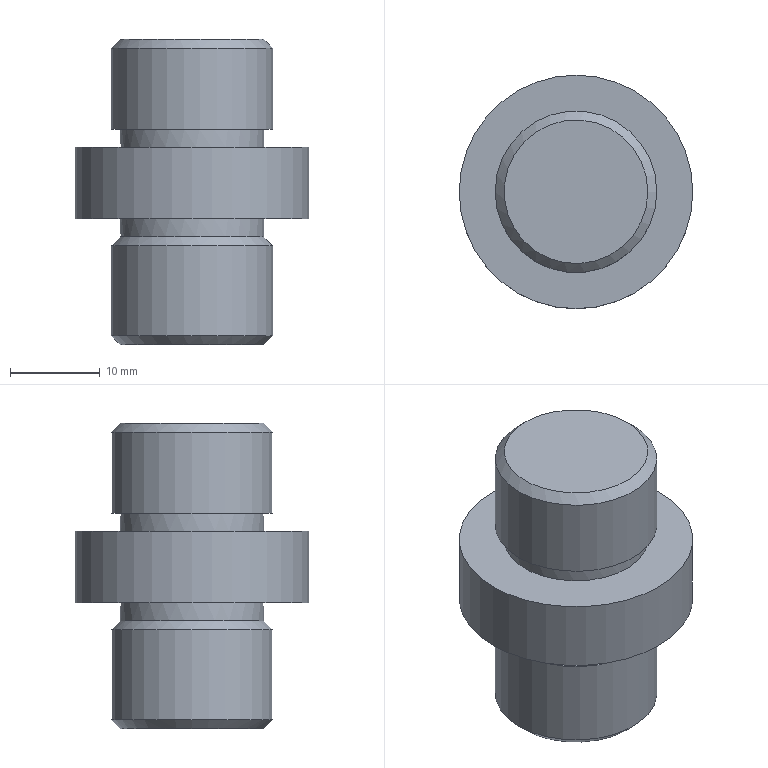Component | NX | DOWEL_PIN | 1 solid | 13 faces | box 26 x 26 x 34 mm | volume 10568 mm3 | plane 5 | cylinder 5 | cone 3 | commonest cylinder face diameters 18 x2 16 x2 26 x1
STEP:
#1=CARTESIAN_POINT('',(0.,0.,0.));
#2=DIRECTION('',(0.,0.,1.));
#3=DIRECTION('',(1.,0.,0.));
#4=AXIS2_PLACEMENT_3D('',#1,#2,#3);
#5=CARTESIAN_POINT('',(-113.,-80.,36.));
#6=VERTEX_POINT('',#5);
#7=CARTESIAN_POINT('',(-105.,-80.,36.));
#8=DIRECTION('',(0.,0.,-1.));
#9=DIRECTION('',(-1.,0.,0.));
#10=AXIS2_PLACEMENT_3D('',#7,#8,#9);
#11=CIRCLE('',#10,8.);
#12=CARTESIAN_POINT('',(-105.,-80.,36.));
#13=DIRECTION('',(0.,0.,-1.));
#14=DIRECTION('',(-1.,0.,0.));
#15=AXIS2_PLACEMENT_3D('',#12,#13,#14);
#16=PLANE('',#15);
#17=CARTESIAN_POINT('',(0.,0.));
#18=DIRECTION('',(1.,0.));
#19=AXIS2_PLACEMENT_2D('',#17,#18);
#20=CIRCLE('',#19,8.);
#21=(GEOMETRIC_REPRESENTATION_CONTEXT(2)PARAMETRIC_REPRESENTATION_CONTEXT()REPRESENTATION_CONTEXT('',''));
#22=DEFINITIONAL_REPRESENTATION('',(#20),#21);
#23=PCURVE('',#16,#22);
#24=CARTESIAN_POINT('',(-105.,-80.,37.));
#25=DIRECTION('',(0.,0.,1.));
#26=DIRECTION('',(1.,0.,0.));
#27=AXIS2_PLACEMENT_3D('',#24,#25,#26);
#28=CONICAL_SURFACE('',#27,9.,0.7854);
#29=CARTESIAN_POINT('',(9.425,-1.));
#30=DIRECTION('',(-1.,0.));
#31=VECTOR('',#30,1.);
#32=LINE('',#29,#31);
#33=(GEOMETRIC_REPRESENTATION_CONTEXT(2)PARAMETRIC_REPRESENTATION_CONTEXT()REPRESENTATION_CONTEXT('',''));
#34=DEFINITIONAL_REPRESENTATION('',(#32),#33);
#35=PCURVE('',#28,#34);
#36=SURFACE_CURVE('',#11,(#23,#35),.PCURVE_S1.);
#37=EDGE_CURVE('',#6,#6,#36,.T.);
#38=ORIENTED_EDGE('',*,*,#37,.T.);
#39=EDGE_LOOP('',(#38));
#40=FACE_BOUND('',#39,.T.);
#41=ADVANCED_FACE('',(#40),#16,.T.);
#42=CARTESIAN_POINT('',(-114.,-80.,37.));
#43=VERTEX_POINT('',#42);
#44=CARTESIAN_POINT('',(-96.,-80.,37.));
#45=VERTEX_POINT('',#44);
#46=CARTESIAN_POINT('',(-105.,-80.,37.));
#47=DIRECTION('',(0.,0.,1.));
#48=DIRECTION('',(-1.,0.,0.));
#49=AXIS2_PLACEMENT_3D('',#46,#47,#48);
#50=CIRCLE('',#49,9.);
#51=CARTESIAN_POINT('',(-105.,-80.,36.));
#52=DIRECTION('',(0.,0.,1.));
#53=DIRECTION('',(1.,0.,0.));
#54=AXIS2_PLACEMENT_3D('',#51,#52,#53);
#55=CYLINDRICAL_SURFACE('',#54,9.);
#56=CARTESIAN_POINT('',(3.142,1.));
#57=DIRECTION('',(1.,0.));
#58=VECTOR('',#57,1.);
#59=LINE('',#56,#58);
#60=(GEOMETRIC_REPRESENTATION_CONTEXT(2)PARAMETRIC_REPRESENTATION_CONTEXT()REPRESENTATION_CONTEXT('',''));
#61=DEFINITIONAL_REPRESENTATION('',(#59),#60);
#62=PCURVE('',#55,#61);
#63=CARTESIAN_POINT('',(3.142,0.));
#64=DIRECTION('',(1.,0.));
#65=VECTOR('',#64,1.);
#66=LINE('',#63,#65);
#67=(GEOMETRIC_REPRESENTATION_CONTEXT(2)PARAMETRIC_REPRESENTATION_CONTEXT()REPRESENTATION_CONTEXT('',''));
#68=DEFINITIONAL_REPRESENTATION('',(#66),#67);
#69=PCURVE('',#28,#68);
#70=SURFACE_CURVE('',#50,(#62,#69),.PCURVE_S1.);
#71=EDGE_CURVE('',#43,#45,#70,.T.);
#72=ORIENTED_EDGE('',*,*,#71,.T.);
#73=CARTESIAN_POINT('',(-96.,-80.,47.));
#74=VERTEX_POINT('',#73);
#75=CARTESIAN_POINT('',(-96.,-80.,37.));
#76=CARTESIAN_POINT('',(-96.,-80.,47.));
#77=B_SPLINE_CURVE_WITH_KNOTS('',1,(#75,#76),.UNSPECIFIED.,.F.,.F.,(2,2),(1.,11.),.PIECEWISE_BEZIER_KNOTS.);
#78=CARTESIAN_POINT('',(6.283,0.));
#79=DIRECTION('',(0.,1.));
#80=VECTOR('',#79,1.);
#81=LINE('',#78,#80);
#82=(GEOMETRIC_REPRESENTATION_CONTEXT(2)PARAMETRIC_REPRESENTATION_CONTEXT()REPRESENTATION_CONTEXT('',''));
#83=DEFINITIONAL_REPRESENTATION('',(#81),#82);
#84=PCURVE('',#55,#83);
#85=CARTESIAN_POINT('',(0.,0.));
#86=DIRECTION('',(0.,1.));
#87=VECTOR('',#86,1.);
#88=LINE('',#85,#87);
#89=(GEOMETRIC_REPRESENTATION_CONTEXT(2)PARAMETRIC_REPRESENTATION_CONTEXT()REPRESENTATION_CONTEXT('',''));
#90=DEFINITIONAL_REPRESENTATION('',(#88),#89);
#91=PCURVE('',#55,#90);
#92=SEAM_CURVE('',#77,(#84,#91),.PCURVE_S1.);
#93=EDGE_CURVE('',#45,#74,#92,.T.);
#94=ORIENTED_EDGE('',*,*,#93,.T.);
#95=CARTESIAN_POINT('',(-105.,-80.,47.));
#96=DIRECTION('',(0.,0.,-1.));
#97=DIRECTION('',(1.,0.,0.));
#98=AXIS2_PLACEMENT_3D('',#95,#96,#97);
#99=CIRCLE('',#98,9.);
#100=CARTESIAN_POINT('',(6.283,11.));
#101=DIRECTION('',(-1.,0.));
#102=VECTOR('',#101,1.);
#103=LINE('',#100,#102);
#104=(GEOMETRIC_REPRESENTATION_CONTEXT(2)PARAMETRIC_REPRESENTATION_CONTEXT()REPRESENTATION_CONTEXT('',''));
#105=DEFINITIONAL_REPRESENTATION('',(#103),#104);
#106=PCURVE('',#55,#105);
#107=CARTESIAN_POINT('',(-105.,-80.,47.));
#108=DIRECTION('',(0.,0.,-1.));
#109=DIRECTION('',(-1.,0.,0.));
#110=AXIS2_PLACEMENT_3D('',#107,#108,#109);
#111=CONICAL_SURFACE('',#110,9.,0.7854);
#112=CARTESIAN_POINT('',(3.142,0.));
#113=DIRECTION('',(1.,0.));
#114=VECTOR('',#113,1.);
#115=LINE('',#112,#114);
#116=(GEOMETRIC_REPRESENTATION_CONTEXT(2)PARAMETRIC_REPRESENTATION_CONTEXT()REPRESENTATION_CONTEXT('',''));
#117=DEFINITIONAL_REPRESENTATION('',(#115),#116);
#118=PCURVE('',#111,#117);
#119=SURFACE_CURVE('',#99,(#106,#118),.PCURVE_S1.);
#120=EDGE_CURVE('',#74,#74,#119,.T.);
#121=ORIENTED_EDGE('',*,*,#120,.T.);
#122=ORIENTED_EDGE('',*,*,#93,.F.);
#123=CARTESIAN_POINT('',(-105.,-80.,37.));
#124=DIRECTION('',(0.,0.,1.));
#125=DIRECTION('',(-1.,0.,0.));
#126=AXIS2_PLACEMENT_3D('',#123,#124,#125);
#127=CIRCLE('',#126,9.);
#128=CARTESIAN_POINT('',(-3.142,1.));
#129=DIRECTION('',(1.,0.));
#130=VECTOR('',#129,1.);
#131=LINE('',#128,#130);
#132=(GEOMETRIC_REPRESENTATION_CONTEXT(2)PARAMETRIC_REPRESENTATION_CONTEXT()REPRESENTATION_CONTEXT('',''));
#133=DEFINITIONAL_REPRESENTATION('',(#131),#132);
#134=PCURVE('',#55,#133);
#135=CARTESIAN_POINT('',(3.142,0.));
#136=DIRECTION('',(1.,0.));
#137=VECTOR('',#136,1.);
#138=LINE('',#135,#137);
#139=(GEOMETRIC_REPRESENTATION_CONTEXT(2)PARAMETRIC_REPRESENTATION_CONTEXT()REPRESENTATION_CONTEXT('',''));
#140=DEFINITIONAL_REPRESENTATION('',(#138),#139);
#141=PCURVE('',#28,#140);
#142=SURFACE_CURVE('',#127,(#134,#141),.PCURVE_S1.);
#143=EDGE_CURVE('',#45,#43,#142,.T.);
#144=ORIENTED_EDGE('',*,*,#143,.T.);
#145=EDGE_LOOP('',(#72,#94,#121,#122,#144));
#146=FACE_BOUND('',#145,.T.);
#147=ADVANCED_FACE('',(#146),#55,.T.);
#148=CARTESIAN_POINT('',(-97.,-80.,50.));
#149=VERTEX_POINT('',#148);
#150=CARTESIAN_POINT('',(-113.,-80.,50.));
#151=VERTEX_POINT('',#150);
#152=CARTESIAN_POINT('',(-105.,-80.,50.));
#153=DIRECTION('',(0.,0.,1.));
#154=DIRECTION('',(-1.,0.,0.));
#155=AXIS2_PLACEMENT_3D('',#152,#153,#154);
#156=CIRCLE('',#155,8.);
#157=CARTESIAN_POINT('',(-105.,-80.,48.));
#158=DIRECTION('',(0.,0.,1.));
#159=DIRECTION('',(1.,0.,0.));
#160=AXIS2_PLACEMENT_3D('',#157,#158,#159);
#161=CYLINDRICAL_SURFACE('',#160,8.);
#162=CARTESIAN_POINT('',(-3.142,2.));
#163=DIRECTION('',(1.,0.));
#164=VECTOR('',#163,1.);
#165=LINE('',#162,#164);
#166=(GEOMETRIC_REPRESENTATION_CONTEXT(2)PARAMETRIC_REPRESENTATION_CONTEXT()REPRESENTATION_CONTEXT('',''));
#167=DEFINITIONAL_REPRESENTATION('',(#165),#166);
#168=PCURVE('',#161,#167);
#169=CARTESIAN_POINT('',(-105.,-80.,50.));
#170=DIRECTION('',(0.,0.,-1.));
#171=DIRECTION('',(-1.,0.,0.));
#172=AXIS2_PLACEMENT_3D('',#169,#170,#171);
#173=PLANE('',#172);
#174=CARTESIAN_POINT('',(8.,0.));
#175=CARTESIAN_POINT('',(8.,-13.856));
#176=CARTESIAN_POINT('',(-4.,-6.928));
#177=CARTESIAN_POINT('',(-16.,-0.));
#178=CARTESIAN_POINT('',(-4.,6.928));
#179=CARTESIAN_POINT('',(8.,13.856));
#180=CARTESIAN_POINT('',(8.,0.));
#181=(BOUNDED_CURVE()B_SPLINE_CURVE(2,(#174,#175,#176,#177,#178,#179,#180),.UNSPECIFIED.,.T.,.F.)B_SPLINE_CURVE_WITH_KNOTS((1,2,2,2,2,1),(-2.094,0.,2.094,4.189,6.283,8.378),.UNSPECIFIED.)CURVE()GEOMETRIC_REPRESENTATION_ITEM()RATIONAL_B_SPLINE_CURVE((1.,0.5,1.,0.5,1.,0.5,1.))REPRESENTATION_ITEM(''));
#182=(GEOMETRIC_REPRESENTATION_CONTEXT(2)PARAMETRIC_REPRESENTATION_CONTEXT()REPRESENTATION_CONTEXT('',''));
#183=DEFINITIONAL_REPRESENTATION('',(#181),#182);
#184=PCURVE('',#173,#183);
#185=SURFACE_CURVE('',#156,(#168,#184),.PCURVE_S1.);
#186=EDGE_CURVE('',#149,#151,#185,.T.);
#187=ORIENTED_EDGE('',*,*,#186,.F.);
#188=CARTESIAN_POINT('',(-97.,-80.,48.));
#189=VERTEX_POINT('',#188);
#190=CARTESIAN_POINT('',(-97.,-80.,48.));
#191=CARTESIAN_POINT('',(-97.,-80.,50.));
#192=B_SPLINE_CURVE_WITH_KNOTS('',1,(#190,#191),.UNSPECIFIED.,.F.,.F.,(2,2),(0.,2.),.PIECEWISE_BEZIER_KNOTS.);
#193=CARTESIAN_POINT('',(0.,0.));
#194=DIRECTION('',(0.,1.));
#195=VECTOR('',#194,1.);
#196=LINE('',#193,#195);
#197=(GEOMETRIC_REPRESENTATION_CONTEXT(2)PARAMETRIC_REPRESENTATION_CONTEXT()REPRESENTATION_CONTEXT('',''));
#198=DEFINITIONAL_REPRESENTATION('',(#196),#197);
#199=PCURVE('',#161,#198);
#200=CARTESIAN_POINT('',(6.283,0.));
#201=DIRECTION('',(0.,1.));
#202=VECTOR('',#201,1.);
#203=LINE('',#200,#202);
#204=(GEOMETRIC_REPRESENTATION_CONTEXT(2)PARAMETRIC_REPRESENTATION_CONTEXT()REPRESENTATION_CONTEXT('',''));
#205=DEFINITIONAL_REPRESENTATION('',(#203),#204);
#206=PCURVE('',#161,#205);
#207=SEAM_CURVE('',#192,(#199,#206),.PCURVE_S1.);
#208=EDGE_CURVE('',#189,#149,#207,.T.);
#209=ORIENTED_EDGE('',*,*,#208,.F.);
#210=CARTESIAN_POINT('',(-105.,-80.,48.));
#211=DIRECTION('',(0.,0.,1.));
#212=DIRECTION('',(1.,0.,0.));
#213=AXIS2_PLACEMENT_3D('',#210,#211,#212);
#214=CIRCLE('',#213,8.);
#215=CARTESIAN_POINT('',(0.,0.));
#216=DIRECTION('',(1.,0.));
#217=VECTOR('',#216,1.);
#218=LINE('',#215,#217);
#219=(GEOMETRIC_REPRESENTATION_CONTEXT(2)PARAMETRIC_REPRESENTATION_CONTEXT()REPRESENTATION_CONTEXT('',''));
#220=DEFINITIONAL_REPRESENTATION('',(#218),#219);
#221=PCURVE('',#161,#220);
#222=CARTESIAN_POINT('',(9.425,-1.));
#223=DIRECTION('',(-1.,0.));
#224=VECTOR('',#223,1.);
#225=LINE('',#222,#224);
#226=(GEOMETRIC_REPRESENTATION_CONTEXT(2)PARAMETRIC_REPRESENTATION_CONTEXT()REPRESENTATION_CONTEXT('',''));
#227=DEFINITIONAL_REPRESENTATION('',(#225),#226);
#228=PCURVE('',#111,#227);
#229=SURFACE_CURVE('',#214,(#221,#228),.PCURVE_S1.);
#230=EDGE_CURVE('',#189,#189,#229,.T.);
#231=ORIENTED_EDGE('',*,*,#230,.T.);
#232=ORIENTED_EDGE('',*,*,#208,.T.);
#233=CARTESIAN_POINT('',(-105.,-80.,50.));
#234=DIRECTION('',(0.,0.,1.));
#235=DIRECTION('',(-1.,0.,0.));
#236=AXIS2_PLACEMENT_3D('',#233,#234,#235);
#237=CIRCLE('',#236,8.);
#238=CARTESIAN_POINT('',(3.142,2.));
#239=DIRECTION('',(1.,0.));
#240=VECTOR('',#239,1.);
#241=LINE('',#238,#240);
#242=(GEOMETRIC_REPRESENTATION_CONTEXT(2)PARAMETRIC_REPRESENTATION_CONTEXT()REPRESENTATION_CONTEXT('',''));
#243=DEFINITIONAL_REPRESENTATION('',(#241),#242);
#244=PCURVE('',#161,#243);
#245=CARTESIAN_POINT('',(8.,0.));
#246=CARTESIAN_POINT('',(8.,-13.856));
#247=CARTESIAN_POINT('',(-4.,-6.928));
#248=CARTESIAN_POINT('',(-16.,-0.));
#249=CARTESIAN_POINT('',(-4.,6.928));
#250=CARTESIAN_POINT('',(8.,13.856));
#251=CARTESIAN_POINT('',(8.,0.));
#252=(BOUNDED_CURVE()B_SPLINE_CURVE(2,(#245,#246,#247,#248,#249,#250,#251),.UNSPECIFIED.,.T.,.F.)B_SPLINE_CURVE_WITH_KNOTS((1,2,2,2,2,1),(-2.094,0.,2.094,4.189,6.283,8.378),.UNSPECIFIED.)CURVE()GEOMETRIC_REPRESENTATION_ITEM()RATIONAL_B_SPLINE_CURVE((1.,0.5,1.,0.5,1.,0.5,1.))REPRESENTATION_ITEM(''));
#253=(GEOMETRIC_REPRESENTATION_CONTEXT(2)PARAMETRIC_REPRESENTATION_CONTEXT()REPRESENTATION_CONTEXT('',''));
#254=DEFINITIONAL_REPRESENTATION('',(#252),#253);
#255=PCURVE('',#173,#254);
#256=SURFACE_CURVE('',#237,(#244,#255),.PCURVE_S1.);
#257=EDGE_CURVE('',#151,#149,#256,.T.);
#258=ORIENTED_EDGE('',*,*,#257,.F.);
#259=EDGE_LOOP('',(#187,#209,#231,#232,#258));
#260=FACE_BOUND('',#259,.T.);
#261=ADVANCED_FACE('',(#260),#161,.T.);
#262=CARTESIAN_POINT('',(-97.,-80.,58.));
#263=VERTEX_POINT('',#262);
#264=CARTESIAN_POINT('',(-105.,-80.,58.));
#265=DIRECTION('',(0.,0.,1.));
#266=DIRECTION('',(1.,0.,0.));
#267=AXIS2_PLACEMENT_3D('',#264,#265,#266);
#268=CIRCLE('',#267,8.);
#269=CARTESIAN_POINT('',(-105.,-80.,58.));
#270=DIRECTION('',(0.,0.,1.));
#271=DIRECTION('',(1.,0.,0.));
#272=AXIS2_PLACEMENT_3D('',#269,#270,#271);
#273=PLANE('',#272);
#274=CARTESIAN_POINT('',(0.,0.));
#275=DIRECTION('',(1.,0.));
#276=AXIS2_PLACEMENT_2D('',#274,#275);
#277=CIRCLE('',#276,8.);
#278=(GEOMETRIC_REPRESENTATION_CONTEXT(2)PARAMETRIC_REPRESENTATION_CONTEXT()REPRESENTATION_CONTEXT('',''));
#279=DEFINITIONAL_REPRESENTATION('',(#277),#278);
#280=PCURVE('',#273,#279);
#281=CARTESIAN_POINT('',(-105.,-80.,58.));
#282=DIRECTION('',(0.,0.,1.));
#283=DIRECTION('',(1.,0.,0.));
#284=AXIS2_PLACEMENT_3D('',#281,#282,#283);
#285=CYLINDRICAL_SURFACE('',#284,8.);
#286=CARTESIAN_POINT('',(0.,0.));
#287=DIRECTION('',(1.,0.));
#288=VECTOR('',#287,1.);
#289=LINE('',#286,#288);
#290=(GEOMETRIC_REPRESENTATION_CONTEXT(2)PARAMETRIC_REPRESENTATION_CONTEXT()REPRESENTATION_CONTEXT('',''));
#291=DEFINITIONAL_REPRESENTATION('',(#289),#290);
#292=PCURVE('',#285,#291);
#293=SURFACE_CURVE('',#268,(#280,#292),.PCURVE_S1.);
#294=EDGE_CURVE('',#263,#263,#293,.T.);
#295=ORIENTED_EDGE('',*,*,#294,.F.);
#296=EDGE_LOOP('',(#295));
#297=FACE_BOUND('',#296,.T.);
#298=CARTESIAN_POINT('',(-92.,-80.,58.));
#299=VERTEX_POINT('',#298);
#300=CARTESIAN_POINT('',(-105.,-80.,58.));
#301=DIRECTION('',(0.,0.,-1.));
#302=DIRECTION('',(1.,0.,0.));
#303=AXIS2_PLACEMENT_3D('',#300,#301,#302);
#304=CIRCLE('',#303,13.);
#305=CARTESIAN_POINT('',(13.,0.));
#306=CARTESIAN_POINT('',(13.,-22.517));
#307=CARTESIAN_POINT('',(-6.5,-11.258));
#308=CARTESIAN_POINT('',(-26.,-0.));
#309=CARTESIAN_POINT('',(-6.5,11.258));
#310=CARTESIAN_POINT('',(13.,22.517));
#311=CARTESIAN_POINT('',(13.,0.));
#312=(BOUNDED_CURVE()B_SPLINE_CURVE(2,(#305,#306,#307,#308,#309,#310,#311),.UNSPECIFIED.,.T.,.F.)B_SPLINE_CURVE_WITH_KNOTS((1,2,2,2,2,1),(-2.094,0.,2.094,4.189,6.283,8.378),.UNSPECIFIED.)CURVE()GEOMETRIC_REPRESENTATION_ITEM()RATIONAL_B_SPLINE_CURVE((1.,0.5,1.,0.5,1.,0.5,1.))REPRESENTATION_ITEM(''));
#313=(GEOMETRIC_REPRESENTATION_CONTEXT(2)PARAMETRIC_REPRESENTATION_CONTEXT()REPRESENTATION_CONTEXT('',''));
#314=DEFINITIONAL_REPRESENTATION('',(#312),#313);
#315=PCURVE('',#273,#314);
#316=CARTESIAN_POINT('',(-105.,-80.,50.));
#317=DIRECTION('',(0.,0.,1.));
#318=DIRECTION('',(1.,0.,0.));
#319=AXIS2_PLACEMENT_3D('',#316,#317,#318);
#320=CYLINDRICAL_SURFACE('',#319,13.);
#321=CARTESIAN_POINT('',(6.283,8.));
#322=DIRECTION('',(-1.,0.));
#323=VECTOR('',#322,1.);
#324=LINE('',#321,#323);
#325=(GEOMETRIC_REPRESENTATION_CONTEXT(2)PARAMETRIC_REPRESENTATION_CONTEXT()REPRESENTATION_CONTEXT('',''));
#326=DEFINITIONAL_REPRESENTATION('',(#324),#325);
#327=PCURVE('',#320,#326);
#328=SURFACE_CURVE('',#304,(#315,#327),.PCURVE_S1.);
#329=EDGE_CURVE('',#299,#299,#328,.T.);
#330=ORIENTED_EDGE('',*,*,#329,.F.);
#331=EDGE_LOOP('',(#330));
#332=FACE_BOUND('',#331,.T.);
#333=ADVANCED_FACE('',(#297,#332),#273,.T.);
#334=ORIENTED_EDGE('',*,*,#257,.T.);
#335=ORIENTED_EDGE('',*,*,#186,.T.);
#336=EDGE_LOOP('',(#334,#335));
#337=FACE_BOUND('',#336,.T.);
#338=CARTESIAN_POINT('',(-92.,-80.,50.));
#339=VERTEX_POINT('',#338);
#340=CARTESIAN_POINT('',(-105.,-80.,50.));
#341=DIRECTION('',(0.,0.,1.));
#342=DIRECTION('',(1.,0.,0.));
#343=AXIS2_PLACEMENT_3D('',#340,#341,#342);
#344=CIRCLE('',#343,13.);
#345=CARTESIAN_POINT('',(-13.,0.));
#346=CARTESIAN_POINT('',(-13.,22.517));
#347=CARTESIAN_POINT('',(6.5,11.258));
#348=CARTESIAN_POINT('',(26.,0.));
#349=CARTESIAN_POINT('',(6.5,-11.258));
#350=CARTESIAN_POINT('',(-13.,-22.517));
#351=CARTESIAN_POINT('',(-13.,0.));
#352=(BOUNDED_CURVE()B_SPLINE_CURVE(2,(#345,#346,#347,#348,#349,#350,#351),.UNSPECIFIED.,.T.,.F.)B_SPLINE_CURVE_WITH_KNOTS((1,2,2,2,2,1),(-2.094,0.,2.094,4.189,6.283,8.378),.UNSPECIFIED.)CURVE()GEOMETRIC_REPRESENTATION_ITEM()RATIONAL_B_SPLINE_CURVE((1.,0.5,1.,0.5,1.,0.5,1.))REPRESENTATION_ITEM(''));
#353=(GEOMETRIC_REPRESENTATION_CONTEXT(2)PARAMETRIC_REPRESENTATION_CONTEXT()REPRESENTATION_CONTEXT('',''));
#354=DEFINITIONAL_REPRESENTATION('',(#352),#353);
#355=PCURVE('',#173,#354);
#356=CARTESIAN_POINT('',(0.,0.));
#357=DIRECTION('',(1.,0.));
#358=VECTOR('',#357,1.);
#359=LINE('',#356,#358);
#360=(GEOMETRIC_REPRESENTATION_CONTEXT(2)PARAMETRIC_REPRESENTATION_CONTEXT()REPRESENTATION_CONTEXT('',''));
#361=DEFINITIONAL_REPRESENTATION('',(#359),#360);
#362=PCURVE('',#320,#361);
#363=SURFACE_CURVE('',#344,(#355,#362),.PCURVE_S1.);
#364=EDGE_CURVE('',#339,#339,#363,.T.);
#365=ORIENTED_EDGE('',*,*,#364,.F.);
#366=EDGE_LOOP('',(#365));
#367=FACE_BOUND('',#366,.T.);
#368=ADVANCED_FACE('',(#337,#367),#173,.T.);
#369=ORIENTED_EDGE('',*,*,#329,.T.);
#370=CARTESIAN_POINT('',(-92.,-80.,50.));
#371=CARTESIAN_POINT('',(-92.,-80.,58.));
#372=B_SPLINE_CURVE_WITH_KNOTS('',1,(#370,#371),.UNSPECIFIED.,.F.,.F.,(2,2),(0.,8.),.PIECEWISE_BEZIER_KNOTS.);
#373=CARTESIAN_POINT('',(0.,0.));
#374=DIRECTION('',(0.,1.));
#375=VECTOR('',#374,1.);
#376=LINE('',#373,#375);
#377=(GEOMETRIC_REPRESENTATION_CONTEXT(2)PARAMETRIC_REPRESENTATION_CONTEXT()REPRESENTATION_CONTEXT('',''));
#378=DEFINITIONAL_REPRESENTATION('',(#376),#377);
#379=PCURVE('',#320,#378);
#380=CARTESIAN_POINT('',(6.283,0.));
#381=DIRECTION('',(0.,1.));
#382=VECTOR('',#381,1.);
#383=LINE('',#380,#382);
#384=(GEOMETRIC_REPRESENTATION_CONTEXT(2)PARAMETRIC_REPRESENTATION_CONTEXT()REPRESENTATION_CONTEXT('',''));
#385=DEFINITIONAL_REPRESENTATION('',(#383),#384);
#386=PCURVE('',#320,#385);
#387=SEAM_CURVE('',#372,(#379,#386),.PCURVE_S1.);
#388=EDGE_CURVE('',#339,#299,#387,.T.);
#389=ORIENTED_EDGE('',*,*,#388,.F.);
#390=ORIENTED_EDGE('',*,*,#364,.T.);
#391=ORIENTED_EDGE('',*,*,#388,.T.);
#392=EDGE_LOOP('',(#369,#389,#390,#391));
#393=FACE_BOUND('',#392,.T.);
#394=ADVANCED_FACE('',(#393),#320,.T.);
#395=CARTESIAN_POINT('',(-97.,-80.,60.));
#396=VERTEX_POINT('',#395);
#397=CARTESIAN_POINT('',(-113.,-80.,60.));
#398=VERTEX_POINT('',#397);
#399=CARTESIAN_POINT('',(-105.,-80.,60.));
#400=DIRECTION('',(0.,0.,1.));
#401=DIRECTION('',(-1.,0.,0.));
#402=AXIS2_PLACEMENT_3D('',#399,#400,#401);
#403=CIRCLE('',#402,8.);
#404=CARTESIAN_POINT('',(-3.142,2.));
#405=DIRECTION('',(1.,0.));
#406=VECTOR('',#405,1.);
#407=LINE('',#404,#406);
#408=(GEOMETRIC_REPRESENTATION_CONTEXT(2)PARAMETRIC_REPRESENTATION_CONTEXT()REPRESENTATION_CONTEXT('',''));
#409=DEFINITIONAL_REPRESENTATION('',(#407),#408);
#410=PCURVE('',#285,#409);
#411=CARTESIAN_POINT('',(-105.,-80.,60.));
#412=DIRECTION('',(0.,0.,-1.));
#413=DIRECTION('',(-1.,0.,0.));
#414=AXIS2_PLACEMENT_3D('',#411,#412,#413);
#415=PLANE('',#414);
#416=CARTESIAN_POINT('',(8.,0.));
#417=CARTESIAN_POINT('',(8.,-13.856));
#418=CARTESIAN_POINT('',(-4.,-6.928));
#419=CARTESIAN_POINT('',(-16.,-0.));
#420=CARTESIAN_POINT('',(-4.,6.928));
#421=CARTESIAN_POINT('',(8.,13.856));
#422=CARTESIAN_POINT('',(8.,0.));
#423=(BOUNDED_CURVE()B_SPLINE_CURVE(2,(#416,#417,#418,#419,#420,#421,#422),.UNSPECIFIED.,.T.,.F.)B_SPLINE_CURVE_WITH_KNOTS((1,2,2,2,2,1),(-2.094,0.,2.094,4.189,6.283,8.378),.UNSPECIFIED.)CURVE()GEOMETRIC_REPRESENTATION_ITEM()RATIONAL_B_SPLINE_CURVE((1.,0.5,1.,0.5,1.,0.5,1.))REPRESENTATION_ITEM(''));
#424=(GEOMETRIC_REPRESENTATION_CONTEXT(2)PARAMETRIC_REPRESENTATION_CONTEXT()REPRESENTATION_CONTEXT('',''));
#425=DEFINITIONAL_REPRESENTATION('',(#423),#424);
#426=PCURVE('',#415,#425);
#427=SURFACE_CURVE('',#403,(#410,#426),.PCURVE_S1.);
#428=EDGE_CURVE('',#396,#398,#427,.T.);
#429=ORIENTED_EDGE('',*,*,#428,.F.);
#430=CARTESIAN_POINT('',(-97.,-80.,58.));
#431=CARTESIAN_POINT('',(-97.,-80.,60.));
#432=B_SPLINE_CURVE_WITH_KNOTS('',1,(#430,#431),.UNSPECIFIED.,.F.,.F.,(2,2),(0.,2.),.PIECEWISE_BEZIER_KNOTS.);
#433=CARTESIAN_POINT('',(0.,0.));
#434=DIRECTION('',(0.,1.));
#435=VECTOR('',#434,1.);
#436=LINE('',#433,#435);
#437=(GEOMETRIC_REPRESENTATION_CONTEXT(2)PARAMETRIC_REPRESENTATION_CONTEXT()REPRESENTATION_CONTEXT('',''));
#438=DEFINITIONAL_REPRESENTATION('',(#436),#437);
#439=PCURVE('',#285,#438);
#440=CARTESIAN_POINT('',(6.283,0.));
#441=DIRECTION('',(0.,1.));
#442=VECTOR('',#441,1.);
#443=LINE('',#440,#442);
#444=(GEOMETRIC_REPRESENTATION_CONTEXT(2)PARAMETRIC_REPRESENTATION_CONTEXT()REPRESENTATION_CONTEXT('',''));
#445=DEFINITIONAL_REPRESENTATION('',(#443),#444);
#446=PCURVE('',#285,#445);
#447=SEAM_CURVE('',#432,(#439,#446),.PCURVE_S1.);
#448=EDGE_CURVE('',#263,#396,#447,.T.);
#449=ORIENTED_EDGE('',*,*,#448,.F.);
#450=ORIENTED_EDGE('',*,*,#294,.T.);
#451=ORIENTED_EDGE('',*,*,#448,.T.);
#452=CARTESIAN_POINT('',(-105.,-80.,60.));
#453=DIRECTION('',(0.,0.,1.));
#454=DIRECTION('',(-1.,0.,0.));
#455=AXIS2_PLACEMENT_3D('',#452,#453,#454);
#456=CIRCLE('',#455,8.);
#457=CARTESIAN_POINT('',(3.142,2.));
#458=DIRECTION('',(1.,0.));
#459=VECTOR('',#458,1.);
#460=LINE('',#457,#459);
#461=(GEOMETRIC_REPRESENTATION_CONTEXT(2)PARAMETRIC_REPRESENTATION_CONTEXT()REPRESENTATION_CONTEXT('',''));
#462=DEFINITIONAL_REPRESENTATION('',(#460),#461);
#463=PCURVE('',#285,#462);
#464=CARTESIAN_POINT('',(8.,0.));
#465=CARTESIAN_POINT('',(8.,-13.856));
#466=CARTESIAN_POINT('',(-4.,-6.928));
#467=CARTESIAN_POINT('',(-16.,-0.));
#468=CARTESIAN_POINT('',(-4.,6.928));
#469=CARTESIAN_POINT('',(8.,13.856));
#470=CARTESIAN_POINT('',(8.,0.));
#471=(BOUNDED_CURVE()B_SPLINE_CURVE(2,(#464,#465,#466,#467,#468,#469,#470),.UNSPECIFIED.,.T.,.F.)B_SPLINE_CURVE_WITH_KNOTS((1,2,2,2,2,1),(-2.094,0.,2.094,4.189,6.283,8.378),.UNSPECIFIED.)CURVE()GEOMETRIC_REPRESENTATION_ITEM()RATIONAL_B_SPLINE_CURVE((1.,0.5,1.,0.5,1.,0.5,1.))REPRESENTATION_ITEM(''));
#472=(GEOMETRIC_REPRESENTATION_CONTEXT(2)PARAMETRIC_REPRESENTATION_CONTEXT()REPRESENTATION_CONTEXT('',''));
#473=DEFINITIONAL_REPRESENTATION('',(#471),#472);
#474=PCURVE('',#415,#473);
#475=SURFACE_CURVE('',#456,(#463,#474),.PCURVE_S1.);
#476=EDGE_CURVE('',#398,#396,#475,.T.);
#477=ORIENTED_EDGE('',*,*,#476,.F.);
#478=EDGE_LOOP('',(#429,#449,#450,#451,#477));
#479=FACE_BOUND('',#478,.T.);
#480=ADVANCED_FACE('',(#479),#285,.T.);
#481=CARTESIAN_POINT('',(-97.,-80.,70.));
#482=VERTEX_POINT('',#481);
#483=CARTESIAN_POINT('',(-105.,-80.,70.));
#484=DIRECTION('',(0.,0.,1.));
#485=DIRECTION('',(1.,0.,0.));
#486=AXIS2_PLACEMENT_3D('',#483,#484,#485);
#487=CIRCLE('',#486,8.);
#488=CARTESIAN_POINT('',(-105.,-80.,70.));
#489=DIRECTION('',(0.,0.,1.));
#490=DIRECTION('',(1.,0.,0.));
#491=AXIS2_PLACEMENT_3D('',#488,#489,#490);
#492=PLANE('',#491);
#493=CARTESIAN_POINT('',(0.,0.));
#494=DIRECTION('',(1.,0.));
#495=AXIS2_PLACEMENT_2D('',#493,#494);
#496=CIRCLE('',#495,8.);
#497=(GEOMETRIC_REPRESENTATION_CONTEXT(2)PARAMETRIC_REPRESENTATION_CONTEXT()REPRESENTATION_CONTEXT('',''));
#498=DEFINITIONAL_REPRESENTATION('',(#496),#497);
#499=PCURVE('',#492,#498);
#500=CARTESIAN_POINT('',(-105.,-80.,69.));
#501=DIRECTION('',(0.,0.,-1.));
#502=DIRECTION('',(-1.,0.,0.));
#503=AXIS2_PLACEMENT_3D('',#500,#501,#502);
#504=CONICAL_SURFACE('',#503,9.,0.7854);
#505=CARTESIAN_POINT('',(9.425,-1.));
#506=DIRECTION('',(-1.,0.));
#507=VECTOR('',#506,1.);
#508=LINE('',#505,#507);
#509=(GEOMETRIC_REPRESENTATION_CONTEXT(2)PARAMETRIC_REPRESENTATION_CONTEXT()REPRESENTATION_CONTEXT('',''));
#510=DEFINITIONAL_REPRESENTATION('',(#508),#509);
#511=PCURVE('',#504,#510);
#512=SURFACE_CURVE('',#487,(#499,#511),.PCURVE_S1.);
#513=EDGE_CURVE('',#482,#482,#512,.T.);
#514=ORIENTED_EDGE('',*,*,#513,.T.);
#515=EDGE_LOOP('',(#514));
#516=FACE_BOUND('',#515,.T.);
#517=ADVANCED_FACE('',(#516),#492,.T.);
#518=ORIENTED_EDGE('',*,*,#476,.T.);
#519=ORIENTED_EDGE('',*,*,#428,.T.);
#520=EDGE_LOOP('',(#518,#519));
#521=FACE_BOUND('',#520,.T.);
#522=CARTESIAN_POINT('',(-96.,-80.,60.));
#523=VERTEX_POINT('',#522);
#524=CARTESIAN_POINT('',(-105.,-80.,60.));
#525=DIRECTION('',(0.,0.,1.));
#526=DIRECTION('',(1.,0.,0.));
#527=AXIS2_PLACEMENT_3D('',#524,#525,#526);
#528=CIRCLE('',#527,9.);
#529=CARTESIAN_POINT('',(-9.,0.));
#530=CARTESIAN_POINT('',(-9.,15.588));
#531=CARTESIAN_POINT('',(4.5,7.794));
#532=CARTESIAN_POINT('',(18.,0.));
#533=CARTESIAN_POINT('',(4.5,-7.794));
#534=CARTESIAN_POINT('',(-9.,-15.588));
#535=CARTESIAN_POINT('',(-9.,0.));
#536=(BOUNDED_CURVE()B_SPLINE_CURVE(2,(#529,#530,#531,#532,#533,#534,#535),.UNSPECIFIED.,.T.,.F.)B_SPLINE_CURVE_WITH_KNOTS((1,2,2,2,2,1),(-2.094,0.,2.094,4.189,6.283,8.378),.UNSPECIFIED.)CURVE()GEOMETRIC_REPRESENTATION_ITEM()RATIONAL_B_SPLINE_CURVE((1.,0.5,1.,0.5,1.,0.5,1.))REPRESENTATION_ITEM(''));
#537=(GEOMETRIC_REPRESENTATION_CONTEXT(2)PARAMETRIC_REPRESENTATION_CONTEXT()REPRESENTATION_CONTEXT('',''));
#538=DEFINITIONAL_REPRESENTATION('',(#536),#537);
#539=PCURVE('',#415,#538);
#540=CARTESIAN_POINT('',(-105.,-80.,60.));
#541=DIRECTION('',(0.,0.,1.));
#542=DIRECTION('',(1.,0.,0.));
#543=AXIS2_PLACEMENT_3D('',#540,#541,#542);
#544=CYLINDRICAL_SURFACE('',#543,9.);
#545=CARTESIAN_POINT('',(0.,0.));
#546=DIRECTION('',(1.,0.));
#547=VECTOR('',#546,1.);
#548=LINE('',#545,#547);
#549=(GEOMETRIC_REPRESENTATION_CONTEXT(2)PARAMETRIC_REPRESENTATION_CONTEXT()REPRESENTATION_CONTEXT('',''));
#550=DEFINITIONAL_REPRESENTATION('',(#548),#549);
#551=PCURVE('',#544,#550);
#552=SURFACE_CURVE('',#528,(#539,#551),.PCURVE_S1.);
#553=EDGE_CURVE('',#523,#523,#552,.T.);
#554=ORIENTED_EDGE('',*,*,#553,.F.);
#555=EDGE_LOOP('',(#554));
#556=FACE_BOUND('',#555,.T.);
#557=ADVANCED_FACE('',(#521,#556),#415,.T.);
#558=CARTESIAN_POINT('',(-96.,-80.,69.));
#559=VERTEX_POINT('',#558);
#560=CARTESIAN_POINT('',(-105.,-80.,69.));
#561=DIRECTION('',(0.,0.,-1.));
#562=DIRECTION('',(1.,0.,0.));
#563=AXIS2_PLACEMENT_3D('',#560,#561,#562);
#564=CIRCLE('',#563,9.);
#565=CARTESIAN_POINT('',(6.283,9.));
#566=DIRECTION('',(-1.,0.));
#567=VECTOR('',#566,1.);
#568=LINE('',#565,#567);
#569=(GEOMETRIC_REPRESENTATION_CONTEXT(2)PARAMETRIC_REPRESENTATION_CONTEXT()REPRESENTATION_CONTEXT('',''));
#570=DEFINITIONAL_REPRESENTATION('',(#568),#569);
#571=PCURVE('',#544,#570);
#572=CARTESIAN_POINT('',(3.142,0.));
#573=DIRECTION('',(1.,0.));
#574=VECTOR('',#573,1.);
#575=LINE('',#572,#574);
#576=(GEOMETRIC_REPRESENTATION_CONTEXT(2)PARAMETRIC_REPRESENTATION_CONTEXT()REPRESENTATION_CONTEXT('',''));
#577=DEFINITIONAL_REPRESENTATION('',(#575),#576);
#578=PCURVE('',#504,#577);
#579=SURFACE_CURVE('',#564,(#571,#578),.PCURVE_S1.);
#580=EDGE_CURVE('',#559,#559,#579,.T.);
#581=ORIENTED_EDGE('',*,*,#580,.T.);
#582=CARTESIAN_POINT('',(-96.,-80.,60.));
#583=CARTESIAN_POINT('',(-96.,-80.,69.));
#584=B_SPLINE_CURVE_WITH_KNOTS('',1,(#582,#583),.UNSPECIFIED.,.F.,.F.,(2,2),(0.,9.),.PIECEWISE_BEZIER_KNOTS.);
#585=CARTESIAN_POINT('',(0.,0.));
#586=DIRECTION('',(0.,1.));
#587=VECTOR('',#586,1.);
#588=LINE('',#585,#587);
#589=(GEOMETRIC_REPRESENTATION_CONTEXT(2)PARAMETRIC_REPRESENTATION_CONTEXT()REPRESENTATION_CONTEXT('',''));
#590=DEFINITIONAL_REPRESENTATION('',(#588),#589);
#591=PCURVE('',#544,#590);
#592=CARTESIAN_POINT('',(6.283,0.));
#593=DIRECTION('',(0.,1.));
#594=VECTOR('',#593,1.);
#595=LINE('',#592,#594);
#596=(GEOMETRIC_REPRESENTATION_CONTEXT(2)PARAMETRIC_REPRESENTATION_CONTEXT()REPRESENTATION_CONTEXT('',''));
#597=DEFINITIONAL_REPRESENTATION('',(#595),#596);
#598=PCURVE('',#544,#597);
#599=SEAM_CURVE('',#584,(#591,#598),.PCURVE_S1.);
#600=EDGE_CURVE('',#523,#559,#599,.T.);
#601=ORIENTED_EDGE('',*,*,#600,.F.);
#602=ORIENTED_EDGE('',*,*,#553,.T.);
#603=ORIENTED_EDGE('',*,*,#600,.T.);
#604=EDGE_LOOP('',(#581,#601,#602,#603));
#605=FACE_BOUND('',#604,.T.);
#606=ADVANCED_FACE('',(#605),#544,.T.);
#607=ORIENTED_EDGE('',*,*,#37,.F.);
#608=CARTESIAN_POINT('',(-113.,-80.,36.));
#609=CARTESIAN_POINT('',(-114.,-80.,37.));
#610=B_SPLINE_CURVE_WITH_KNOTS('',1,(#608,#609),.UNSPECIFIED.,.F.,.F.,(2,2),(-1.414,0.),.PIECEWISE_BEZIER_KNOTS.);
#611=CARTESIAN_POINT('',(9.425,0.));
#612=DIRECTION('',(0.,1.));
#613=VECTOR('',#612,1.);
#614=LINE('',#611,#613);
#615=(GEOMETRIC_REPRESENTATION_CONTEXT(2)PARAMETRIC_REPRESENTATION_CONTEXT()REPRESENTATION_CONTEXT('',''));
#616=DEFINITIONAL_REPRESENTATION('',(#614),#615);
#617=PCURVE('',#28,#616);
#618=CARTESIAN_POINT('',(3.142,0.));
#619=DIRECTION('',(0.,1.));
#620=VECTOR('',#619,1.);
#621=LINE('',#618,#620);
#622=(GEOMETRIC_REPRESENTATION_CONTEXT(2)PARAMETRIC_REPRESENTATION_CONTEXT()REPRESENTATION_CONTEXT('',''));
#623=DEFINITIONAL_REPRESENTATION('',(#621),#622);
#624=PCURVE('',#28,#623);
#625=SEAM_CURVE('',#610,(#617,#624),.PCURVE_S1.);
#626=EDGE_CURVE('',#6,#43,#625,.T.);
#627=ORIENTED_EDGE('',*,*,#626,.T.);
#628=ORIENTED_EDGE('',*,*,#143,.F.);
#629=ORIENTED_EDGE('',*,*,#71,.F.);
#630=ORIENTED_EDGE('',*,*,#626,.F.);
#631=EDGE_LOOP('',(#607,#627,#628,#629,#630));
#632=FACE_BOUND('',#631,.T.);
#633=ADVANCED_FACE('',(#632),#28,.T.);
#634=ORIENTED_EDGE('',*,*,#230,.F.);
#635=CARTESIAN_POINT('',(-97.,-80.,48.));
#636=CARTESIAN_POINT('',(-96.,-80.,47.));
#637=B_SPLINE_CURVE_WITH_KNOTS('',1,(#635,#636),.UNSPECIFIED.,.F.,.F.,(2,2),(-1.414,0.),.PIECEWISE_BEZIER_KNOTS.);
#638=CARTESIAN_POINT('',(9.425,0.));
#639=DIRECTION('',(0.,1.));
#640=VECTOR('',#639,1.);
#641=LINE('',#638,#640);
#642=(GEOMETRIC_REPRESENTATION_CONTEXT(2)PARAMETRIC_REPRESENTATION_CONTEXT()REPRESENTATION_CONTEXT('',''));
#643=DEFINITIONAL_REPRESENTATION('',(#641),#642);
#644=PCURVE('',#111,#643);
#645=CARTESIAN_POINT('',(3.142,0.));
#646=DIRECTION('',(0.,1.));
#647=VECTOR('',#646,1.);
#648=LINE('',#645,#647);
#649=(GEOMETRIC_REPRESENTATION_CONTEXT(2)PARAMETRIC_REPRESENTATION_CONTEXT()REPRESENTATION_CONTEXT('',''));
#650=DEFINITIONAL_REPRESENTATION('',(#648),#649);
#651=PCURVE('',#111,#650);
#652=SEAM_CURVE('',#637,(#644,#651),.PCURVE_S1.);
#653=EDGE_CURVE('',#189,#74,#652,.T.);
#654=ORIENTED_EDGE('',*,*,#653,.T.);
#655=ORIENTED_EDGE('',*,*,#120,.F.);
#656=ORIENTED_EDGE('',*,*,#653,.F.);
#657=EDGE_LOOP('',(#634,#654,#655,#656));
#658=FACE_BOUND('',#657,.T.);
#659=ADVANCED_FACE('',(#658),#111,.T.);
#660=ORIENTED_EDGE('',*,*,#513,.F.);
#661=CARTESIAN_POINT('',(-97.,-80.,70.));
#662=CARTESIAN_POINT('',(-96.,-80.,69.));
#663=B_SPLINE_CURVE_WITH_KNOTS('',1,(#661,#662),.UNSPECIFIED.,.F.,.F.,(2,2),(-1.414,0.),.PIECEWISE_BEZIER_KNOTS.);
#664=CARTESIAN_POINT('',(9.425,0.));
#665=DIRECTION('',(0.,1.));
#666=VECTOR('',#665,1.);
#667=LINE('',#664,#666);
#668=(GEOMETRIC_REPRESENTATION_CONTEXT(2)PARAMETRIC_REPRESENTATION_CONTEXT()REPRESENTATION_CONTEXT('',''));
#669=DEFINITIONAL_REPRESENTATION('',(#667),#668);
#670=PCURVE('',#504,#669);
#671=CARTESIAN_POINT('',(3.142,0.));
#672=DIRECTION('',(0.,1.));
#673=VECTOR('',#672,1.);
#674=LINE('',#671,#673);
#675=(GEOMETRIC_REPRESENTATION_CONTEXT(2)PARAMETRIC_REPRESENTATION_CONTEXT()REPRESENTATION_CONTEXT('',''));
#676=DEFINITIONAL_REPRESENTATION('',(#674),#675);
#677=PCURVE('',#504,#676);
#678=SEAM_CURVE('',#663,(#670,#677),.PCURVE_S1.);
#679=EDGE_CURVE('',#482,#559,#678,.T.);
#680=ORIENTED_EDGE('',*,*,#679,.T.);
#681=ORIENTED_EDGE('',*,*,#580,.F.);
#682=ORIENTED_EDGE('',*,*,#679,.F.);
#683=EDGE_LOOP('',(#660,#680,#681,#682));
#684=FACE_BOUND('',#683,.T.);
#685=ADVANCED_FACE('',(#684),#504,.T.);
#686=CLOSED_SHELL('',(#41,#147,#261,#333,#368,#394,#480,#517,#557,#606,#633,#659,#685));
#687=MANIFOLD_SOLID_BREP('',#686);
#688=(LENGTH_UNIT()NAMED_UNIT(*)SI_UNIT(.MILLI.,.METRE.));
#689=UNCERTAINTY_MEASURE_WITH_UNIT(LENGTH_MEASURE(0.000005),#688,'','');
#690=(NAMED_UNIT(*)PLANE_ANGLE_UNIT()SI_UNIT($,.RADIAN.));
#691=(NAMED_UNIT(*)SI_UNIT($,.STERADIAN.)SOLID_ANGLE_UNIT());
#692=(GEOMETRIC_REPRESENTATION_CONTEXT(3)GLOBAL_UNCERTAINTY_ASSIGNED_CONTEXT((#689))GLOBAL_UNIT_ASSIGNED_CONTEXT((#688,#690,#691))REPRESENTATION_CONTEXT('',''));
#693=ADVANCED_BREP_SHAPE_REPRESENTATION('',(#4,#687),#692);